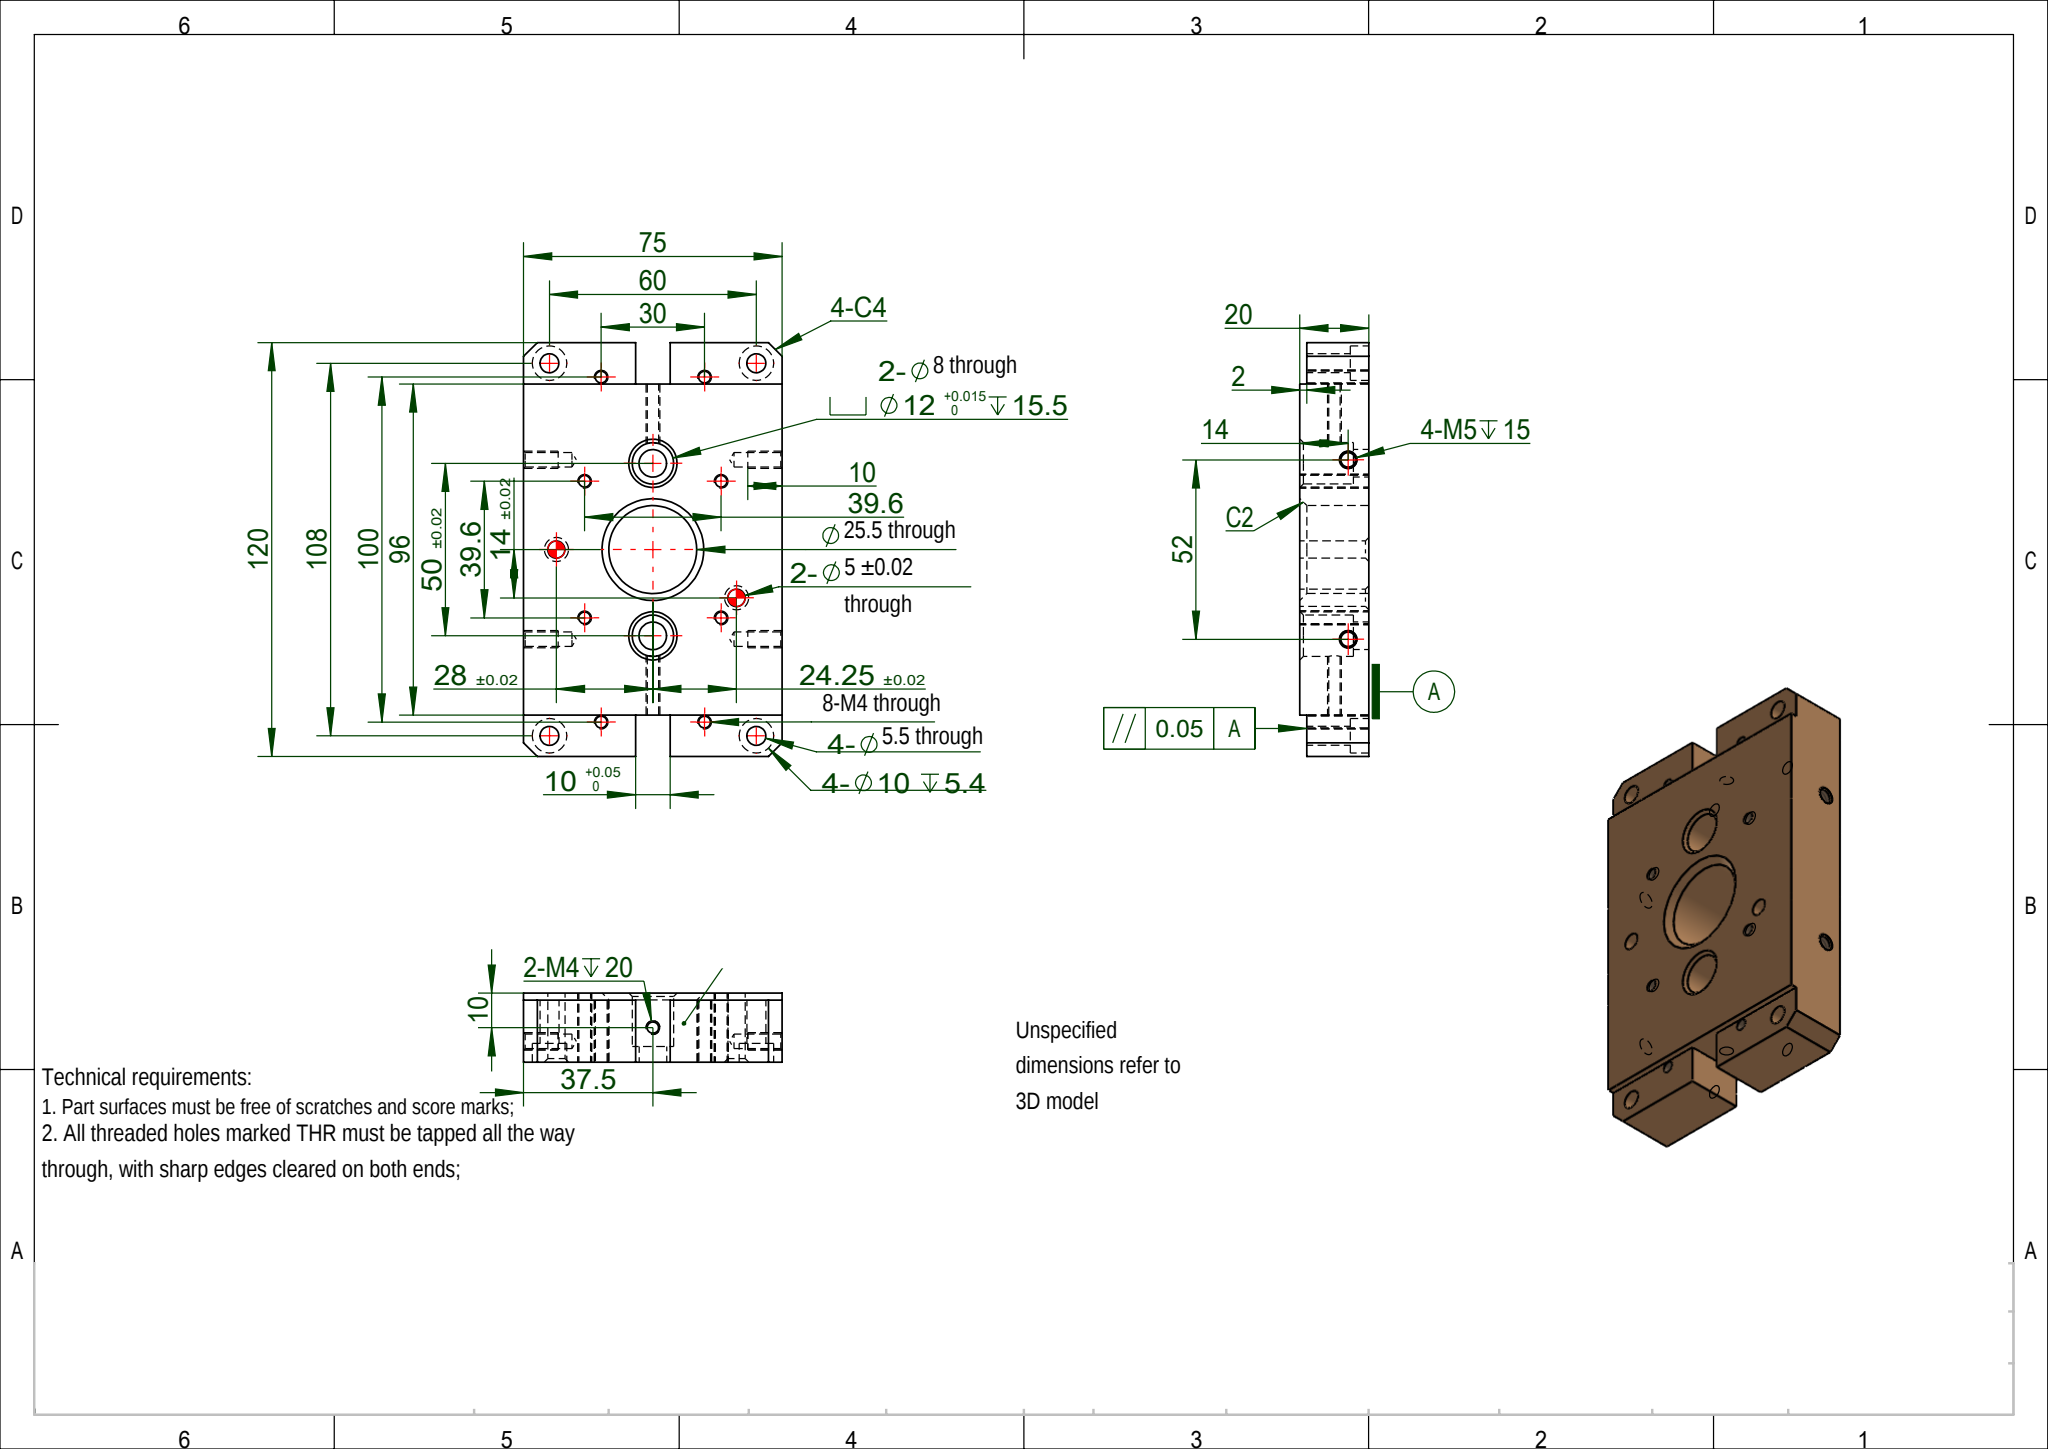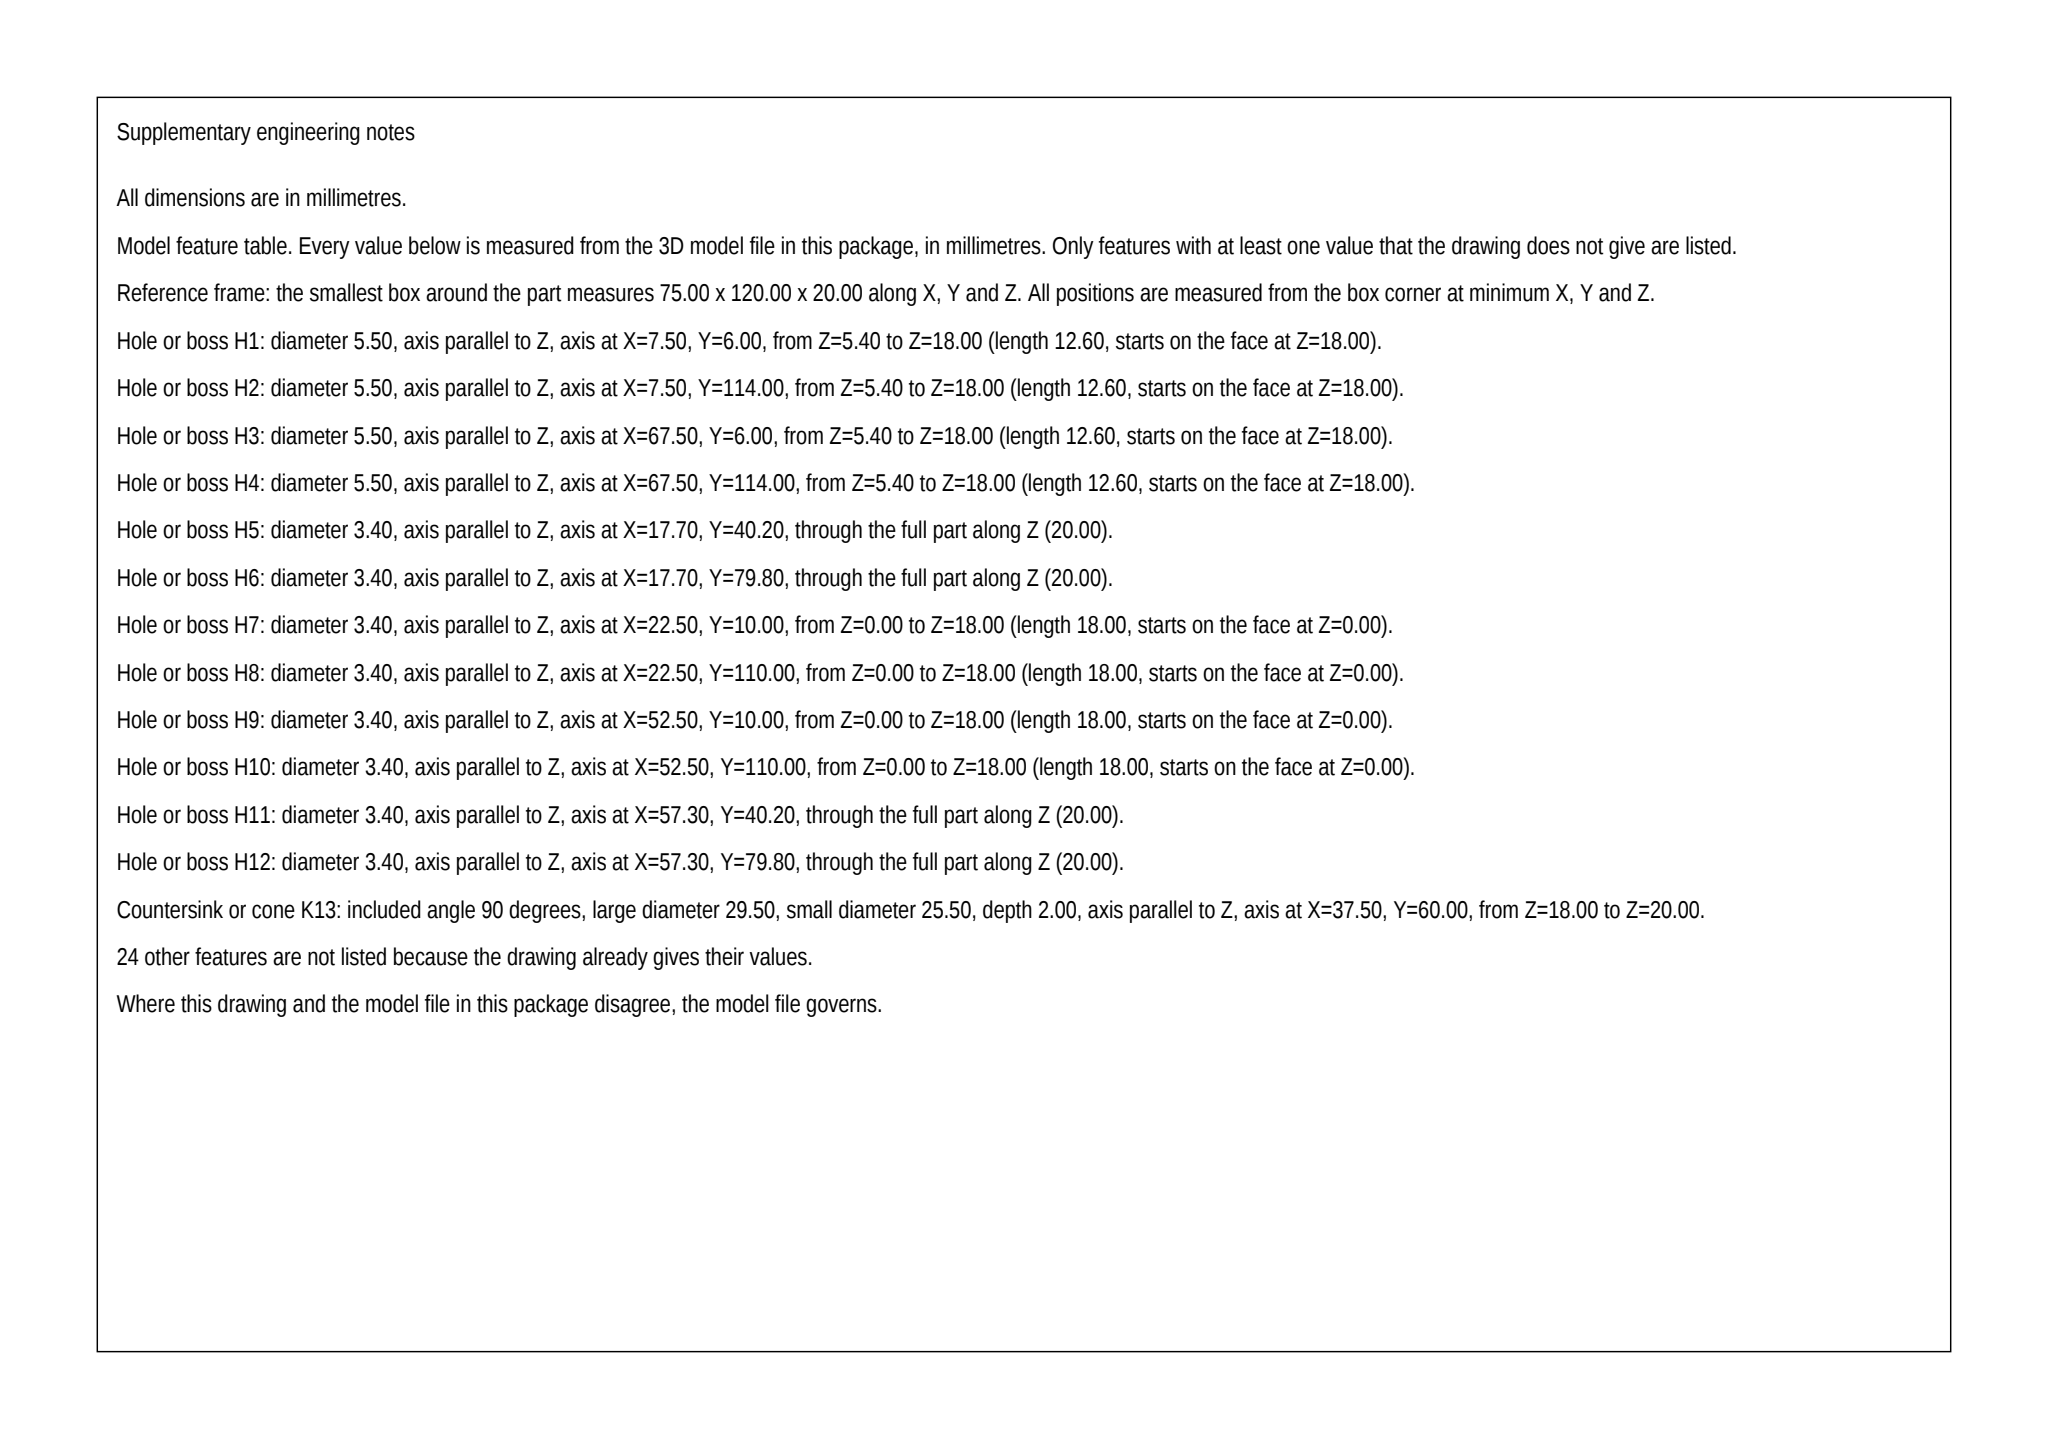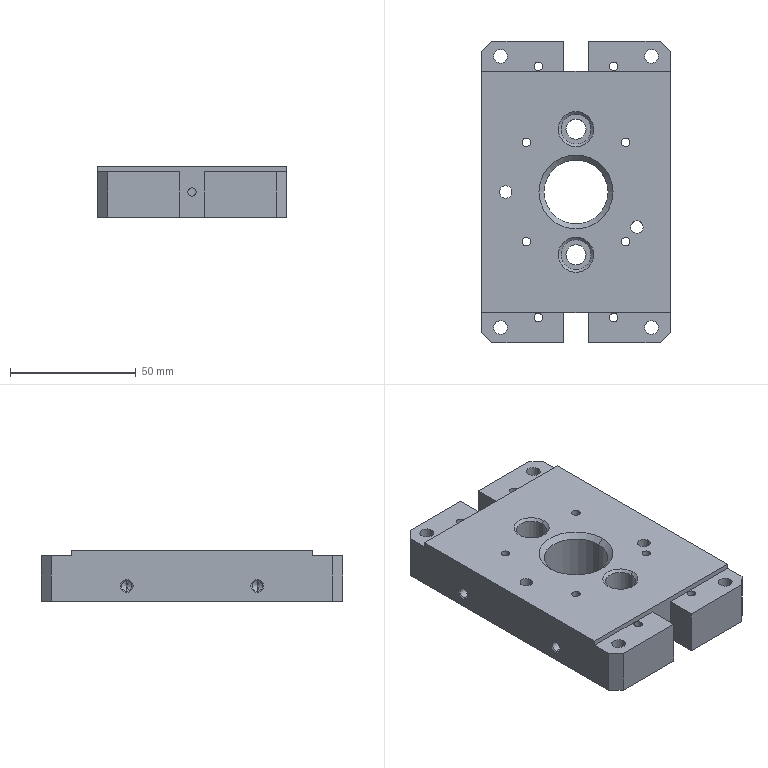Part | SolidWorks | mm | 1 solid | 112 faces | box 75 x 120 x 20 mm | volume 150950 mm3 | cylinder 58 | plane 28 | cone 26 | commonest cylinder face diameters 3.4 x16 4.2 x8 10 x8 5.5 x8 3.3 x4 12 x4 5 x4 8 x4
build123d program:
from build123d import *

# Parameters (mm, degrees)
SKETCH1_W                                       = 75
SKETCH1_H                                       = 120
BOSS_EXTRUDE1_DEPTH                             = 20
CHAMFER1_SIZE                                   = 4
M5_HEX_SOCKET_HEAD_CAP_SCREW_CBORE1_D           = 5.5
M5_HEX_SOCKET_HEAD_CAP_SCREW_CBORE1_CBORE_D     = 10
M5_HEX_SOCKET_HEAD_CAP_SCREW_CBORE1_CBORE_DEPTH = 5.4
SKETCH16_W                                      = 2
SKETCH16_H                                      = 20
CUT_EXTRUDE3_DEPTH                              = 99.107
SKETCH17_R                                      = 1.7
SKETCH17_R_2                                    = 2.5
CUT_EXTRUDE4_DEPTH                              = 20
CHAMFER2_SIZE                                   = 1
SKETCH19_R                                      = 12.75
CUT_EXTRUDE5_DEPTH                              = 74.527
M5_TAPPED_HOLE1_AT_2_COUNT                      = 2
M5_TAPPED_HOLE1_AT_2_PITCH                      = 52
CHAMFER3_SIZE                                   = 2
SKETCH24_R                                      = 1.7
CUT_EXTRUDE6_DEPTH                              = 20
SKETCH25_W                                      = 10
SKETCH25_H                                      = 36
CUT_EXTRUDE7_DEPTH                              = 12
SKETCH26_R                                      = 4
CUT_EXTRUDE8_DEPTH                              = 20
CHAMFER4_SIZE                                   = 1
SKETCH27_R                                      = 6
CUT_EXTRUDE9_DEPTH                              = 15.5
CHAMFER5_SIZE                                   = 1


with BuildPart() as part:
    # Sketch1 → Boss-Extrude1 (new body)
    with BuildSketch(Plane.XY):
        Rectangle(SKETCH1_W, SKETCH1_H)
    extrude(amount=BOSS_EXTRUDE1_DEPTH)

    # Chamfer1
    chamfer1_edges = [part.edges().sort_by_distance(p)[0] for p in [
        (-37.5, 60, 10),
        (37.5, 60, 10),
        (37.5, -60, 10),
        (-37.5, -60, 10),
    ]]
    chamfer(chamfer1_edges, length=CHAMFER1_SIZE)

    # M5 Hex Socket Head Cap Screw CBORE1 (through all)
    with Locations(Plane(origin=(0, 0, 0), x_dir=(-1, 0, 0), z_dir=(0, 0, -1))):
        with Locations((30, -54), (-30, -54)):
            m5_hex_socket_head_cap_screw_cbore1 = CounterBoreHole(M5_HEX_SOCKET_HEAD_CAP_SCREW_CBORE1_D / 2, M5_HEX_SOCKET_HEAD_CAP_SCREW_CBORE1_CBORE_D / 2, M5_HEX_SOCKET_HEAD_CAP_SCREW_CBORE1_CBORE_DEPTH)

    # Sketch16 → Cut-Extrude3 (cut, through all)
    with BuildSketch(Plane.ZY.offset(37.5)):
        with Locations((19, 58)):
            Rectangle(SKETCH16_W, SKETCH16_H)
        with Locations((19, -58)):
            Rectangle(SKETCH16_W, SKETCH16_H)
    extrude(amount=-CUT_EXTRUDE3_DEPTH, mode=Mode.SUBTRACT)

    # Mirror1: M5 Hex Socket Head Cap Screw CBORE1 across plane
    add(m5_hex_socket_head_cap_screw_cbore1.mirror(Plane.ZX), mode=Mode.SUBTRACT)

    # Sketch17 → Cut-Extrude4 (cut)
    with BuildSketch(Plane.XY.offset(20)):
        with Locations((-19.799, 19.799)):
            Circle(SKETCH17_R)
        with Locations((-28, 0)):
            Circle(SKETCH17_R_2)
        with Locations((19.799, 19.799)):
            Circle(SKETCH17_R)
        with Locations((19.799, -19.799)):
            Circle(SKETCH17_R)
        with Locations((-19.799, -19.799)):
            Circle(SKETCH17_R)
        with Locations((24.249, -14)):
            Circle(SKETCH17_R_2)
    extrude(amount=-CUT_EXTRUDE4_DEPTH, mode=Mode.SUBTRACT)

    # Chamfer2
    chamfer2_edges = [part.edges().sort_by_distance(p)[0] for p in [
        (-30.5, 0, 0),
        (21.749, -14, 0),
    ]]
    chamfer(chamfer2_edges, length=CHAMFER2_SIZE)

    # Sketch19 → Cut-Extrude5 (cut, through all)
    with BuildSketch(Plane(origin=(0, 0, 0), x_dir=(-1, 0, 0), z_dir=(0, 0, -1))):
        Circle(SKETCH19_R)
    extrude(amount=-CUT_EXTRUDE5_DEPTH, mode=Mode.SUBTRACT)

    # Sketch21 → M5 Tapped Hole1 (revolve, cut)
    with BuildSketch(Plane(origin=(-37.5, 26, 6), x_dir=(0, 0, 1), z_dir=(0, 1, 0))):
        Polygon((0, 0), (0, 15.262), (2.1, 14), (2.1, 0.425), (2.525, 0), align=None)
    m5_tapped_hole1 = revolve(axis=Axis((-43.85, 26, 6), (1, 0, 0)), mode=Mode.SUBTRACT)

    # M5 Tapped Hole1 at 2: M5 Tapped Hole1 ×2
    with Locations(*[(0, -i * M5_TAPPED_HOLE1_AT_2_PITCH, 0) for i in range(1, M5_TAPPED_HOLE1_AT_2_COUNT)]):
        add(m5_tapped_hole1, mode=Mode.SUBTRACT)

    # Mirror2: M5 Tapped Hole1 across plane
    add(m5_tapped_hole1.mirror(Plane(origin=(0, 0, 0), x_dir=(0, 0, 1), z_dir=(1, 0, 0))), mode=Mode.SUBTRACT)

    # Mirror2 copy 1 sketch → Mirror2 copy 1 (revolve, cut)
    with BuildSketch(Plane(origin=(37.5, -26, 6), x_dir=(0, 0, 1), z_dir=(0, 1, 0))):
        Polygon((0, 0), (0, -15.262), (2.1, -14), (2.1, -0.425), (2.525, 0), align=None)
    revolve(axis=Axis((43.85, -26, 6), (1, 0, 0)), mode=Mode.SUBTRACT)

    # Chamfer3
    chamfer3_edges = [part.edges().sort_by_distance(p)[0] for p in [
        (12.75, 0, 20),
    ]]
    chamfer(chamfer3_edges, length=CHAMFER3_SIZE)

    # Sketch24 → Cut-Extrude6 (cut)
    with BuildSketch(Plane(origin=(0, 0, 0), x_dir=(-1, 0, 0), z_dir=(0, 0, -1))):
        with Locations((-15, 50)):
            Circle(SKETCH24_R)
        with Locations((15, 50)):
            Circle(SKETCH24_R)
        with Locations((-15, -50)):
            Circle(SKETCH24_R)
        with Locations((15, -50)):
            Circle(SKETCH24_R)
    extrude(amount=-CUT_EXTRUDE6_DEPTH, mode=Mode.SUBTRACT)

    # Sketch25 → Cut-Extrude7 (cut)
    with BuildSketch(Plane.XZ.offset(60)):
        Rectangle(SKETCH25_W, SKETCH25_H)
    cut_extrude7 = extrude(amount=-CUT_EXTRUDE7_DEPTH, mode=Mode.SUBTRACT)

    # Mirror3: Cut-Extrude7 across plane
    add(cut_extrude7.mirror(Plane.ZX), mode=Mode.SUBTRACT)

    # Sketch26 → Cut-Extrude8 (cut)
    with BuildSketch(Plane.XY.offset(20)):
        with Locations((0, 25)):
            Circle(SKETCH26_R)
        with Locations((0, -25)):
            Circle(SKETCH26_R)
    extrude(amount=-CUT_EXTRUDE8_DEPTH, mode=Mode.SUBTRACT)

    # Chamfer4
    chamfer4_edges = [part.edges().sort_by_distance(p)[0] for p in [
        (-4, 25, 20),
        (-4, -25, 20),
    ]]
    chamfer(chamfer4_edges, length=CHAMFER4_SIZE)

    # Sketch27 → Cut-Extrude9 (cut)
    with BuildSketch(Plane.XY.offset(20)):
        with Locations((0, -25)):
            Circle(SKETCH27_R)
    cut_extrude9 = extrude(amount=-CUT_EXTRUDE9_DEPTH, mode=Mode.SUBTRACT)

    # Mirror4: Cut-Extrude9 across plane
    add(cut_extrude9.mirror(Plane.ZX), mode=Mode.SUBTRACT)

    # Chamfer5
    chamfer5_edges = [part.edges().sort_by_distance(p)[0] for p in [
        (-6, -25, 20),
        (-6, 25, 20),
    ]]
    chamfer(chamfer5_edges, length=CHAMFER5_SIZE)

    # Sketch28 → M4 Tapped Hole1 (revolve, cut)
    with BuildSketch(Plane(origin=(0, -48, 10), x_dir=(0, 0, -1), z_dir=(1, 0, 0))):
        Polygon((0, 0), (0, 26.991), (1.65, 26), (1.65, 0), align=None)
    m4_tapped_hole1 = revolve(axis=Axis((0, -54.35, 10), (0, 1, 0)), mode=Mode.SUBTRACT)

    # Mirror5: M4 Tapped Hole1 across plane
    add(m4_tapped_hole1.mirror(Plane.ZX), mode=Mode.SUBTRACT)


solid = part.part